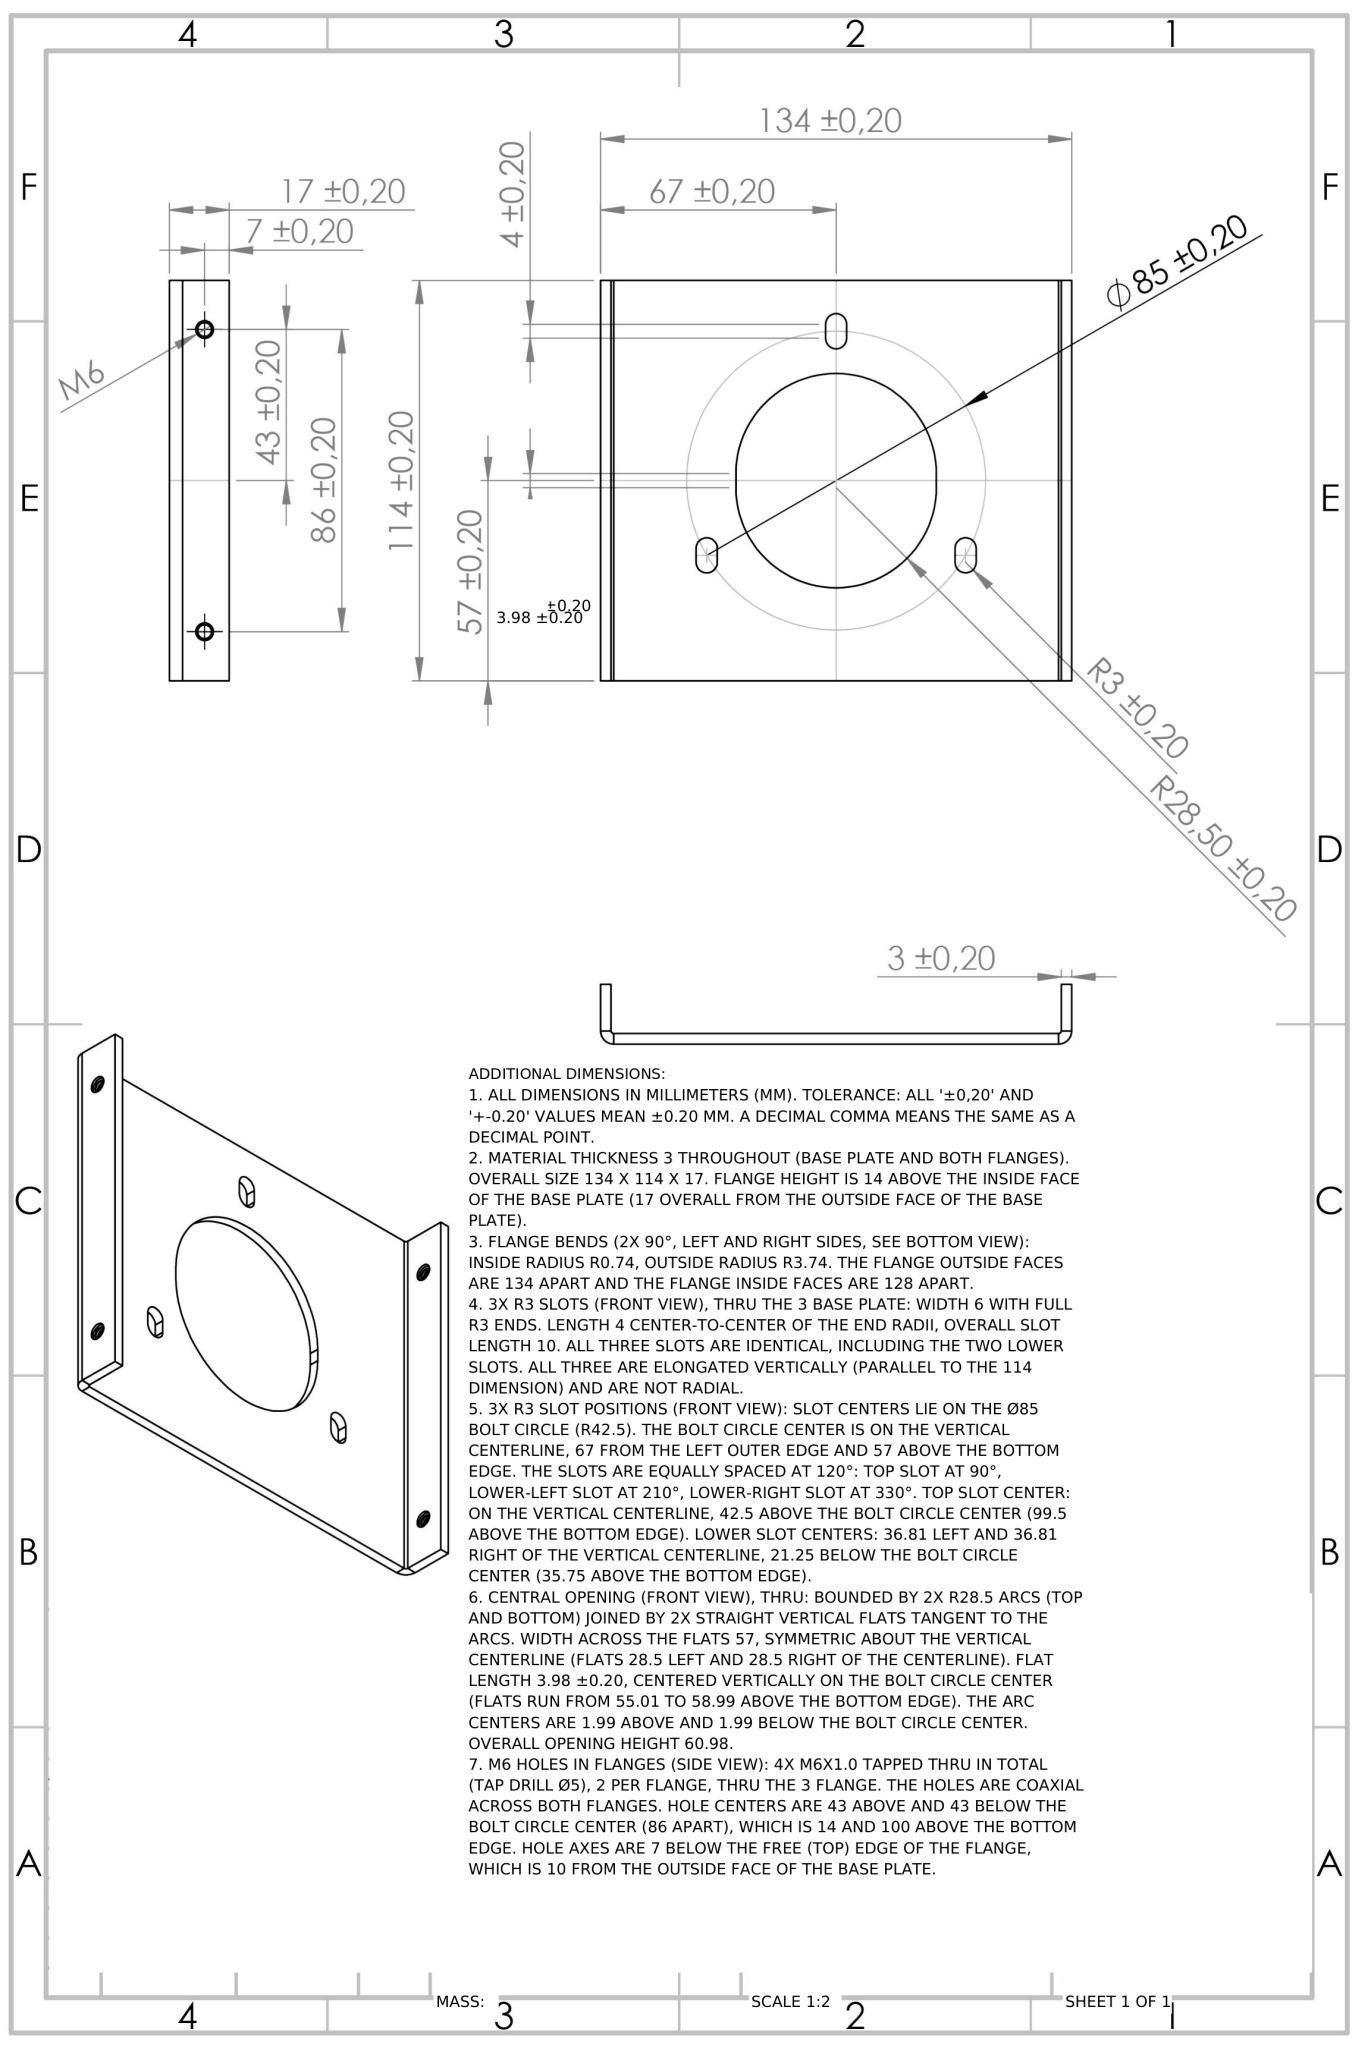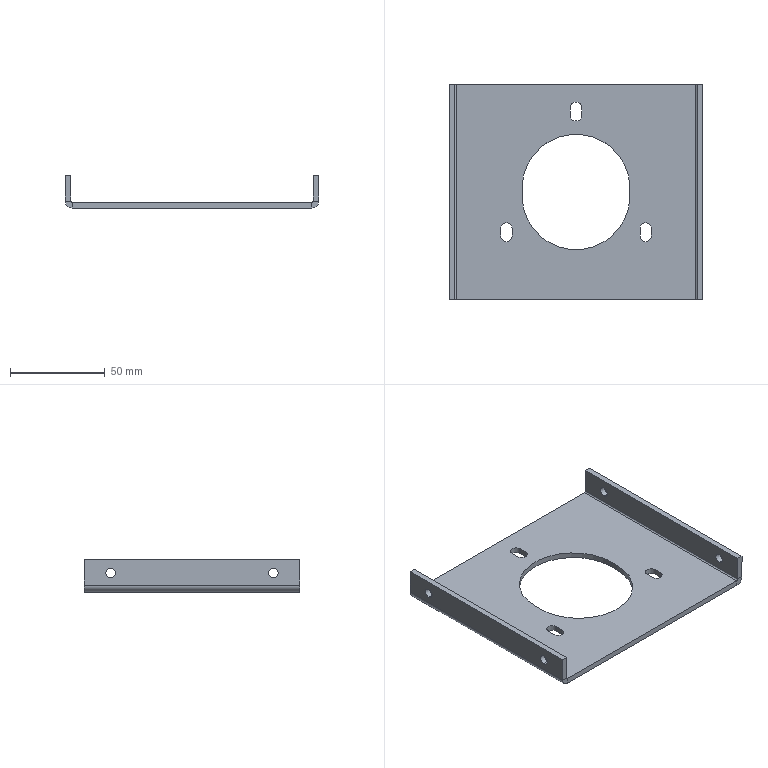Part | NX | mm | 1 solid | 46 faces | box 134 x 114 x 17 mm | volume 45705 mm3 | plane 26 | cylinder 20 | commonest cylinder face diameters 5 x8 7.473 x2 1.473 x2 6.009 x2 57 x2 5.995 x2 6.006 x2